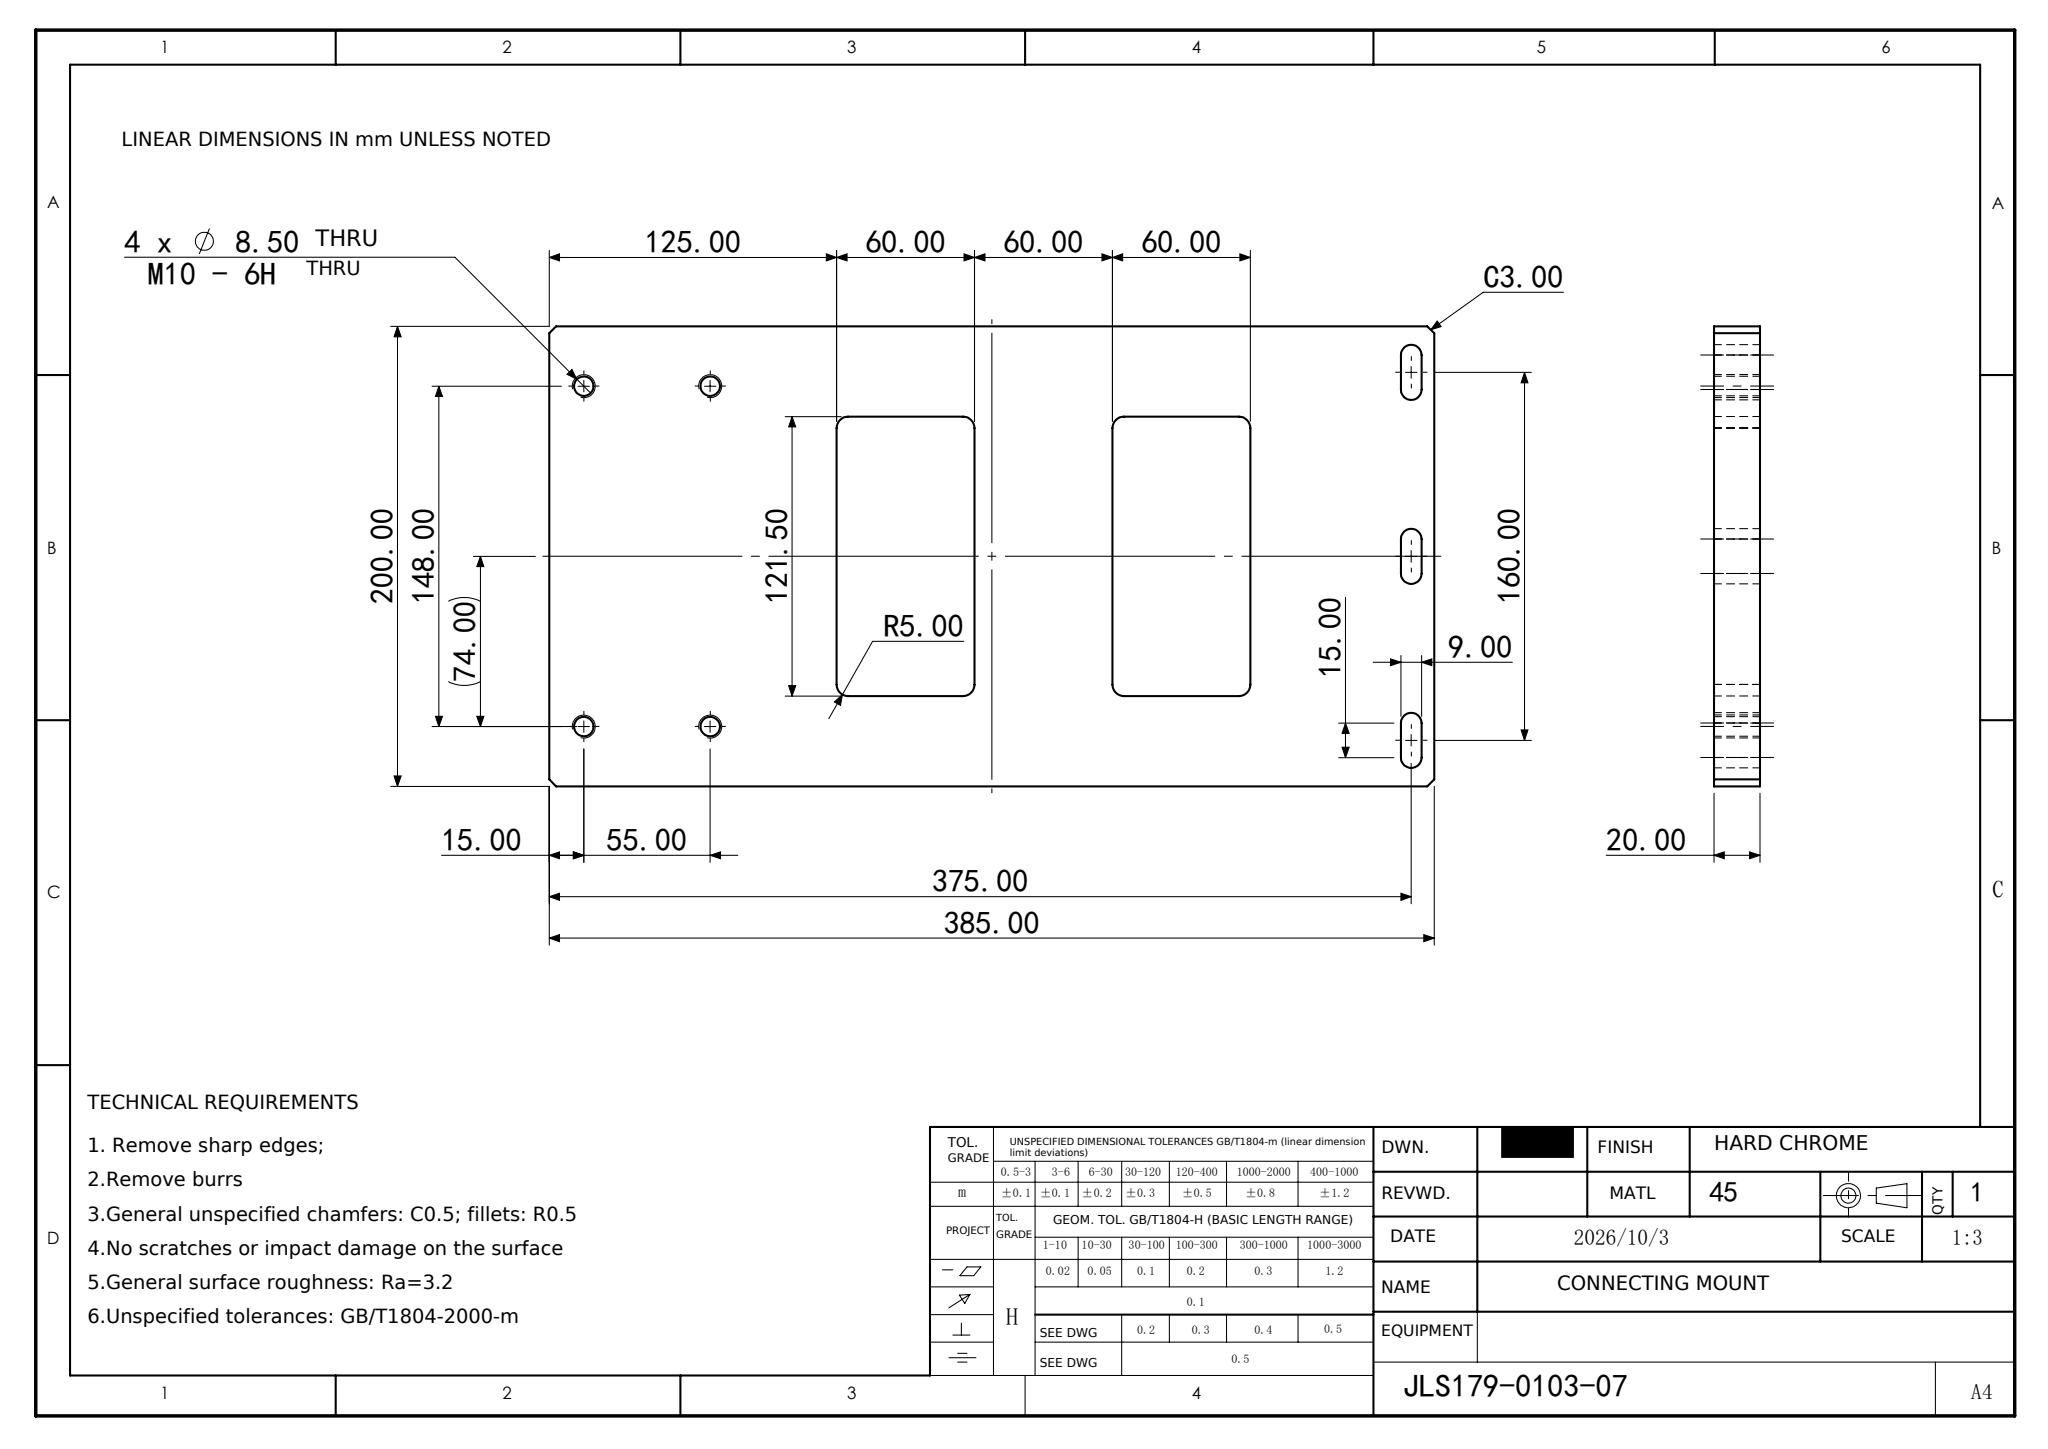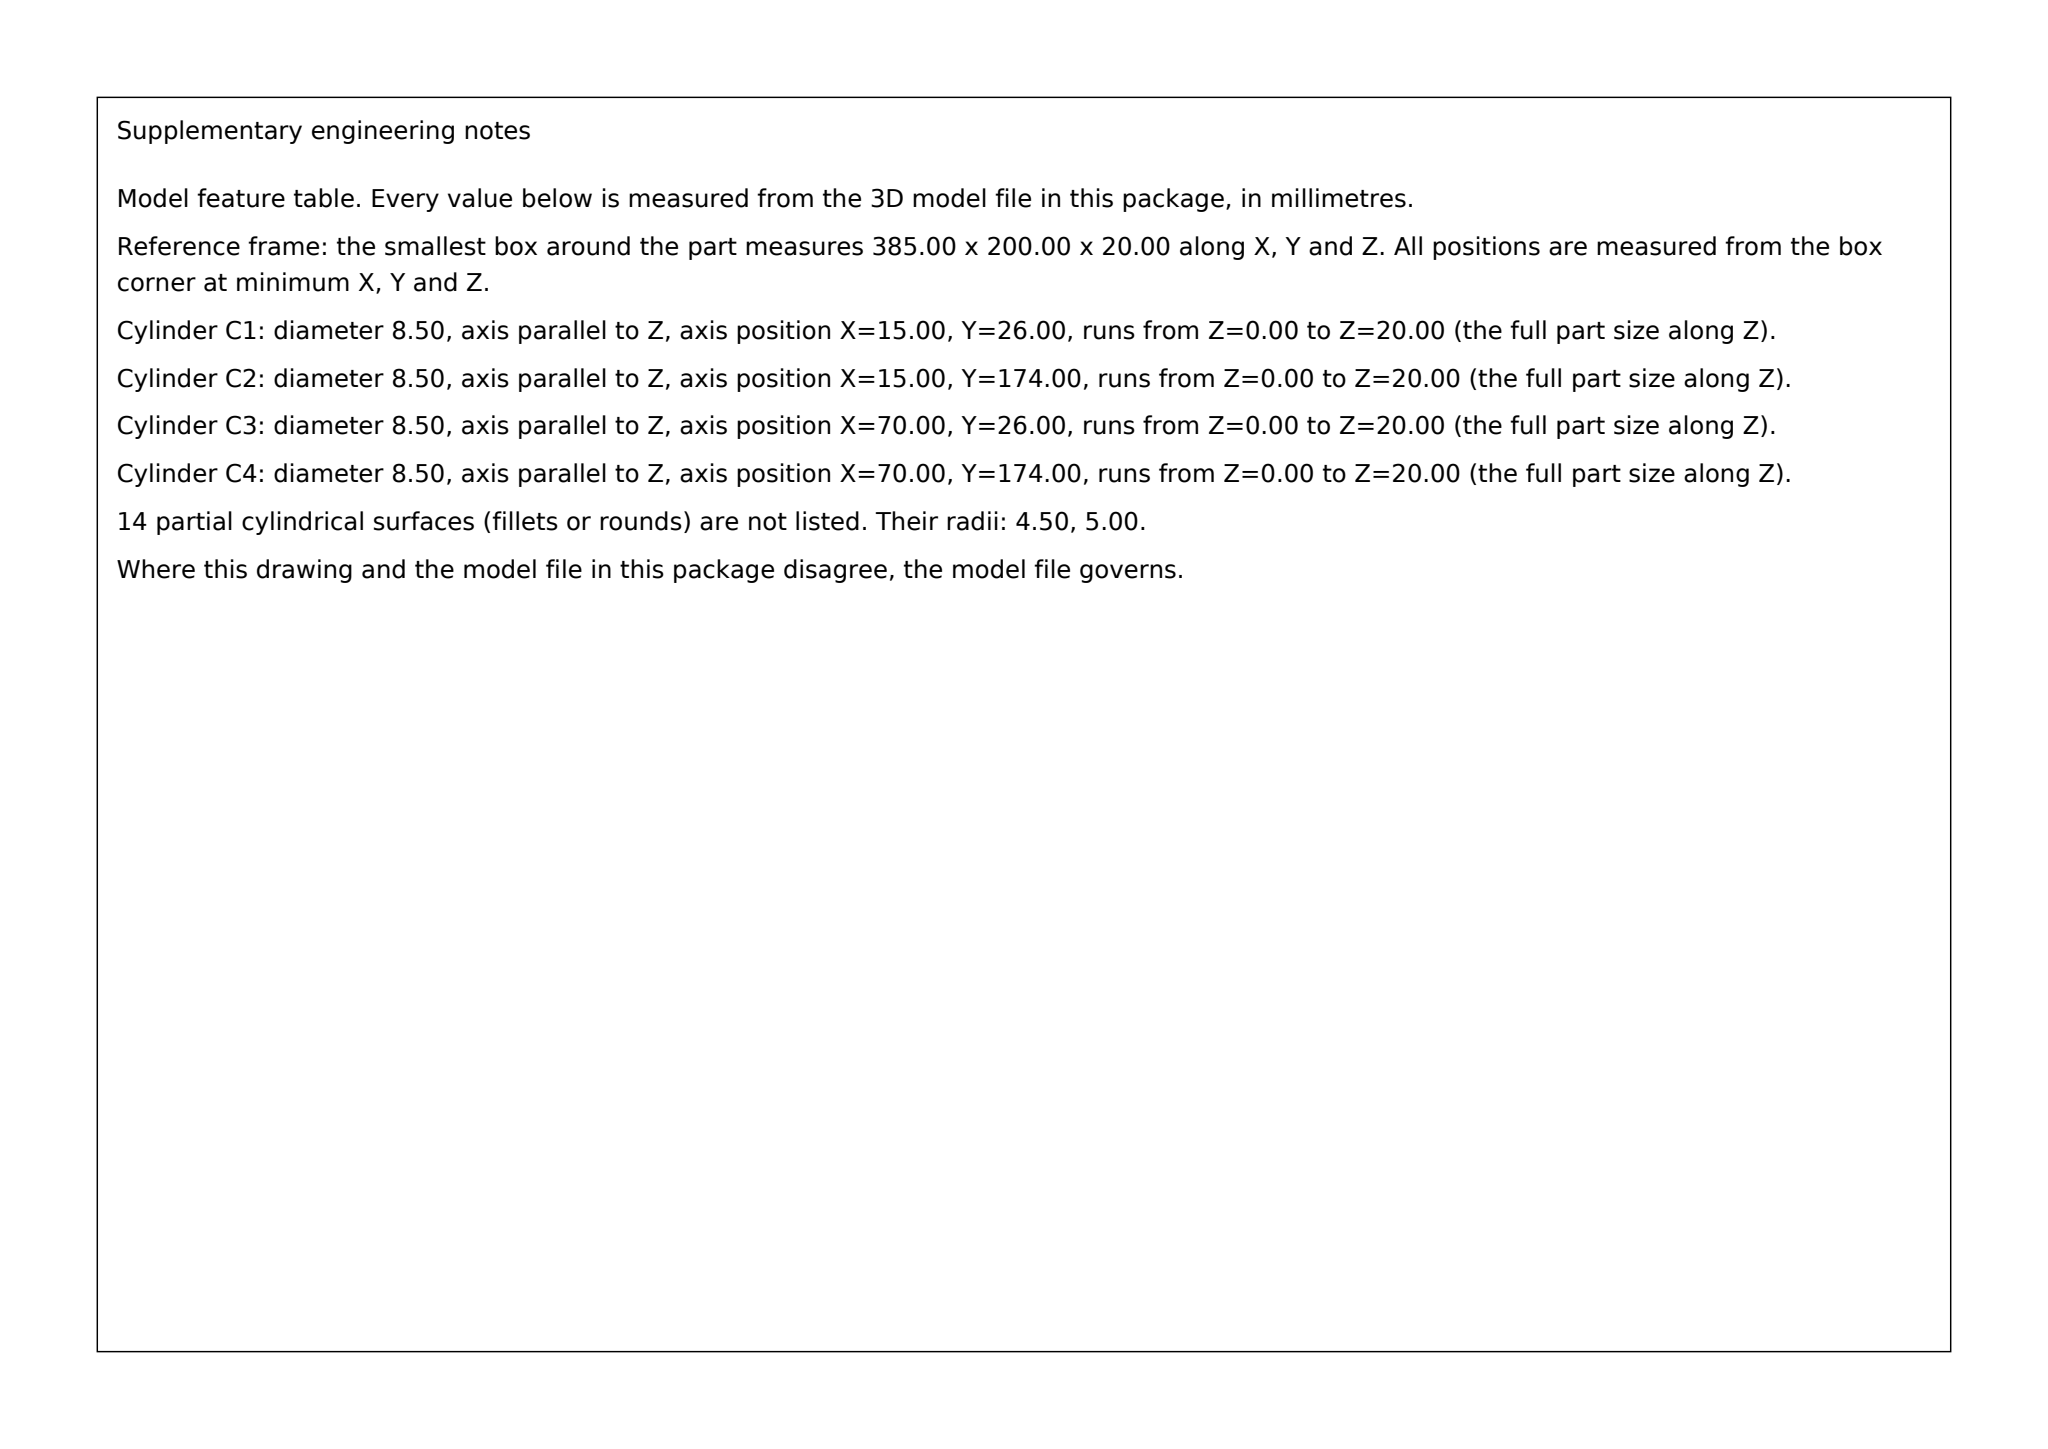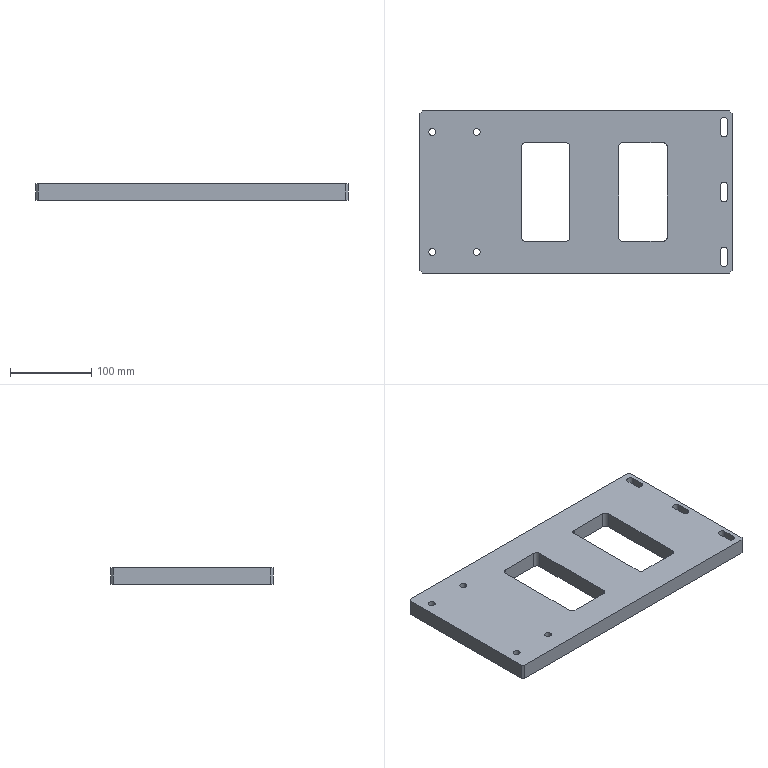Part | SolidWorks | mm | material 45 | 1 solid | 46 faces | box 385 x 200 x 20 mm | volume 1232432 mm3 | plane 24 | cylinder 22 | commonest cylinder face diameters 8.5 x8 10 x8 9 x6
build123d program:
from build123d import *

# Parameters (mm, degrees)
SKETCH1_W           = 385
SKETCH1_H           = 200
BOSS_EXTRUDE1_DEPTH = 20
CHAMFER1_SIZE       = 3
CUT_EXTRUDE1_DEPTH  = 218.845
M10_TAPPED_HOLE1_D  = 8.5
SKETCH5_W           = 60
SKETCH5_H           = 121.504
CUT_EXTRUDE2_DEPTH  = 218.845
FILLET1_R           = 5


with BuildPart() as part:
    # Sketch1 → Boss-Extrude1 (new body)
    with BuildSketch(Plane.XY):
        Rectangle(SKETCH1_W, SKETCH1_H)
    extrude(amount=BOSS_EXTRUDE1_DEPTH)

    # Chamfer1
    chamfer1_edges = [part.edges().sort_by_distance(p)[0] for p in [
        (192.5, -100, 10),
        (-192.5, -100, 10),
        (-192.5, 100, 10),
        (192.5, 100, 10),
    ]]
    chamfer(chamfer1_edges, length=CHAMFER1_SIZE)

    # Sketch2 → Cut-Extrude1 (cut, through all)
    with BuildSketch(Plane(origin=(0, 0, 0), x_dir=(-1, 0, 0), z_dir=(0, 0, -1))):
        with BuildLine():
            Line((-187, -7.5), (-187, 7.5))
            ThreePointArc((-187, 7.5), (-182.5, 12), (-178, 7.5))
            Line((-178, 7.5), (-178, -7.5))
            ThreePointArc((-178, -7.5), (-182.5, -12), (-187, -7.5))
        make_face()
        with BuildLine():
            Line((-187, 72.5), (-187, 87.5))
            ThreePointArc((-187, 87.5), (-182.5, 92), (-178, 87.5))
            Line((-178, 87.5), (-178, 72.5))
            ThreePointArc((-178, 72.5), (-182.5, 68), (-187, 72.5))
        make_face()
        with BuildLine():
            Line((-187, -72.5), (-187, -87.5))
            ThreePointArc((-187, -87.5), (-182.5, -92), (-178, -87.5))
            Line((-178, -87.5), (-178, -72.5))
            ThreePointArc((-178, -72.5), (-182.5, -68), (-187, -72.5))
        make_face()
    extrude(amount=-CUT_EXTRUDE1_DEPTH, mode=Mode.SUBTRACT)

    # M10 Tapped Hole1 (through all)
    with Locations(Plane.XY.offset(20)):
        with Locations((-122.5, 74), (-177.5, 74), (-122.5, -74), (-177.5, -74)):
            Hole(M10_TAPPED_HOLE1_D / 2)

    # Sketch5 → Cut-Extrude2 (cut, through all)
    with BuildSketch(Plane(origin=(0, 0, 0), x_dir=(-1, 0, 0), z_dir=(0, 0, -1))):
        with Locations((-82.5, 0)):
            Rectangle(SKETCH5_W, SKETCH5_H)
        with Locations((37.5, 0)):
            Rectangle(SKETCH5_W, SKETCH5_H)
    extrude(amount=-CUT_EXTRUDE2_DEPTH, mode=Mode.SUBTRACT)

    # Fillet1
    fillet1_edges = [part.edges().sort_by_distance(p)[0] for p in [
        (52.5, 60.752, 10),
        (52.5, -60.752, 10),
        (112.5, -60.752, 10),
        (112.5, 60.752, 10),
        (-67.5, 60.752, 10),
        (-67.5, -60.752, 10),
        (-7.5, -60.752, 10),
        (-7.5, 60.752, 10),
    ]]
    fillet(fillet1_edges, radius=FILLET1_R)


solid = part.part